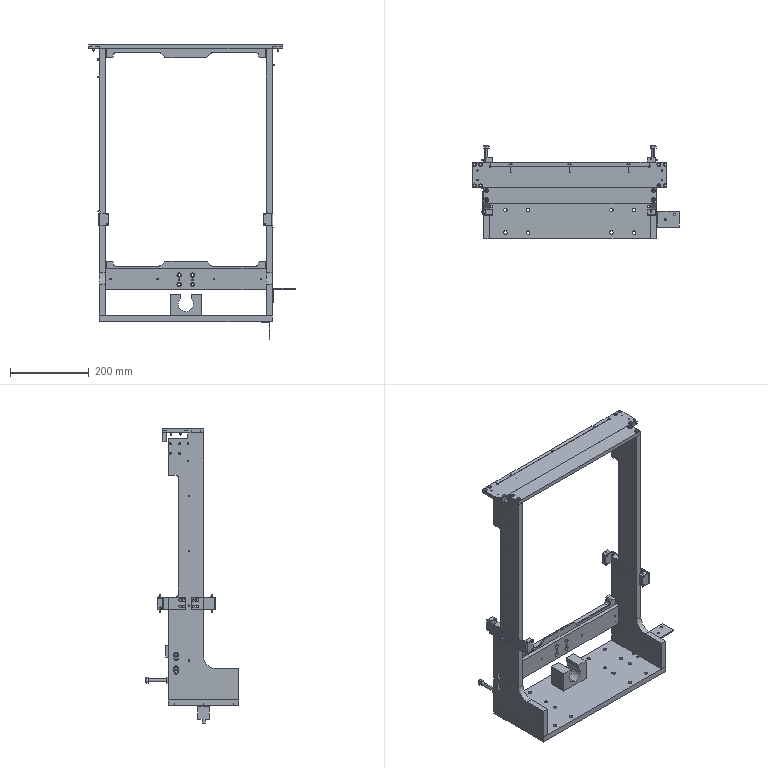Assembly | SolidWorks | mm | 33 component files | 33 solids | 1082 faces | box 526.5 x 239 x 749 mm | volume 4007622 mm3 | cylinder 498 | plane 446 | cone 118 | sphere 20 | commonest cylinder face diameters 5 x69 6.6 x50 11 x47 10 x42 9 x40 3.3 x32 3 x32 5.5 x24
Bill of materials:
30-20A | 1 |  | Flat rectangular plate with many through-holes in a symmetric pattern.
30-24A | 1 |  | Rectangular block with a U-shaped slot: a round bore runs through the block and opens to the top face through a straight-sided slot.
30-27A | 1 |  | Tall, thin, roughly L-shaped plate: a long vertical upright with a short foot at the bottom joined by a rounded inside corner, a long relief cut along one edge, and scattered holes.
30-28A | 1 |  | Tall, thin, roughly L-shaped plate almost identical to unnamed part, with a different hole pattern: smaller holes at the top and two extra small holes in the foot.
30-29A | 1 |  | Long, thin, flat bar with stepped ends: a raised tab at each end and hole groups at both ends, including slot-like or notched openings at the edges.
30-30A | 1 |  | Plain, long, thin rectangular flat bar with two through-holes at each end.
30-32A | 1 |  | Long, narrow, bar-shaped plate with a shaped lower edge: a down-stepped foot at each end, a wide central lobe with angled sides, and three evenly spaced round holes along the upper area.
30-41A | 1 |  | Bent L-shaped bracket with a radiused bend: a longer flange with two holes and a shorter flange at right angles with two holes.
30-49A | 4 |  | Thin L-shaped bracket with a radiused bend: one flange has two elongated slots, the other has two round holes.
30-51A | 1 |  | Small bent bracket with a radiused bend: a horizontal flange with two round holes and a vertical flange ending in a narrower tab at the bottom.
KFQAPP3-P3.00-L4-B4.0 | 8 |  | Solid cylindrical pin with one hemispherical (domed) end and one flat end.
KFQAPP4-P4.00-L4-B4.0 | 2 |  | Solid cylindrical pin with one hemispherical (domed) end and one flat end.
30-31A | 1 |  | Long, thin rectangular flat bar with a pattern of small and larger through holes across its broad face, plus two holes in one end face.
30-33A | 1 |  | Long rectangular bar with a stepped top profile: a raised tab at each end with a small hooked notch, lower recessed runs, and a raised center section with angled transitions; two through holes in the center region.
Q20EBanner | 2 |  | Rectangular block body with two through holes near opposite corners, an angled cylindrical protrusion leaving one corner, a small cylindrical stub on one face, and two shallow raised rectangular pads on one side face.
Q20NRBanner | 2 |  | Rectangular block body with two through holes, an angled cylindrical protrusion from a chamfered corner, and small raised pads on one side face; close to a mirrored or reoriented version of the previous block part.
NUT_K8 | 2 |  | Hexagonal nut-like body with a central round bore and chamfered corners on both faces.
UST8_60b | 2 |  | Hex-head bolt-like part: a hexagonal head with a short cylindrical boss on its outer face and a long plain cylindrical shank ending in a chamfered tip.
Mates:
1. coincident | 30-20A-1 face at (-869.208, 12.908, 39.188) dir (0, 0, 1) | 30-28A-1 face at (-444.208, -167.092, 39.188) dir (0, 0, -1)
2. coincident | 30-20A-1 face at (-429.208, -167.092, 24.188) dir (1, 0, 0) | 30-28A-1 face at (-429.208, -107.092, 149.188) dir (1, 0, 0)
3. coincident | 30-20A-1 face at (-869.208, -167.092, 24.188) dir (0, -1, 0) | 30-28A-1 face at (-444.208, -167.092, 39.188) dir (0, -1, 0)
4. coincident | 30-20A-1 face at (-869.208, 12.908, 39.188) dir (0, 0, 1) | 30-27A-1 face at (-869.208, -167.092, 39.188) dir (0, 0, -1)
5. coincident | 30-20A-1 face at (-869.208, -167.092, 24.188) dir (-1, 0, 0) | 30-27A-1 face at (-869.208, -107.092, 149.188) dir (-1, 0, 0)
6. coincident | 30-20A-1 face at (-869.208, 12.908, 24.188) dir (0, 1, 0) | 30-27A-1 face at (-869.208, 12.908, 39.188) dir (0, 1, 0)
7. coincident | 30-20A-1 plane at (-649.208, -77.092, 39.188) dir (1, 0, 0) | 30-24A-1 plane at (-649.208, -37.092, 66.188) dir (-1, 0, 0)
8. coincident | 30-20A-1 plane at (-649.208, -77.092, 39.188) dir (1, 0, 0) | assembly plane at (-649.208, 11.408, 176.688) dir (1, 0, 0)
9. distance | 30-28A-1 face at (-444.208, 12.908, 39.188) dir (0, 1, 0) | assembly face at (-224.366, 15.085, 546.382) dir (0, 1, 0)
10. distance | 30-28A-1 face at (-444.208, 12.908, 39.188) dir (0, 1, 0) | UST8_60-1/UST8_60b-1 face at (-859.001, 4.408, 90.956) dir (0, -1, 0)
11. concentric | 30-27A-1 face at (-861.708, 12.908, 89.188) dir (0, 1, 0) r 4.05 | UST8_60-1/UST8_60b-1 face at (-861.708, 4.408, 89.188) dir (0, 1, 0) r 4
12. concentric | 30-28A-1 face at (-436.708, 12.908, 89.188) dir (0, 1, 0) r 4.05 | UST8_60-2/UST8_60b-1 face at (-436.708, 4.408, 89.188) dir (0, 1, 0) r 4
13. distance | 30-28A-1 face at (-444.208, 12.908, 39.188) dir (0, 1, 0) | UST8_60-2/NUT_K8-1 face at (-436.708, 12.908, 89.188) dir (0, -1, 0)
14. coincident | 30-28A-1 face at (-429.208, -107.092, 149.188) dir (1, 0, 0) | assembly face at (-419.208, -53.092, 330.922) dir (-1, 0, 0)
15. coincident | 30-28A-1 face at (-444.208, -77.092, 719.188) dir (0, -1, 0) | assembly face at (-417.208, -51.092, 330.922) dir (0, 1, 0)
16. concentric | 30-27A-1 face at (-861.708, -45.092, 719.188) dir (0, 0, 1) r 2.5 | 30-30A-1 face at (-861.708, -45.092, 729.188) dir (0, 0, 1) r 5.5
17. concentric | 30-27A-1 face at (-861.708, -69.092, 719.188) dir (0, 0, 1) r 2.5 | 30-30A-1 face at (-861.708, -69.092, 729.188) dir (0, 0, 1) r 5.5
18. coincident | 30-27A-1 face at (-869.208, 12.908, 719.188) dir (0, 0, 1) | 30-30A-1 face at (-869.208, -77.092, 719.188) dir (0, 0, -1)
19. concentric | 30-27A-1 face at (-854.208, -37.592, 692.188) dir (-1, 0, 0) r 1.5 | KFQAPP3-P3.00-L4-B4.0-1 face at (-908.289, -37.592, 692.188) dir (-1, 0, 0) r 1.5
20. concentric | 30-27A-1 face at (-854.208, -37.592, 647.188) dir (-1, 0, 0) r 1.5 | KFQAPP3-P3.00-L4-B4.0-2 face at (-908.289, -37.592, 647.188) dir (-1, 0, 0) r 1.5
21. coincident | KFQAPP3-P3.00-L4-B4.0-2 face at (-865.208, -37.996, 648.632) dir (1, 0, 0) | KFQAPP3-P3.00-L4-B4.0-1 face at (-865.208, -37.952, 693.644) dir (1, 0, 0)
22. concentric | 30-28A-1 face at (-444.208, 7.908, 679.188) dir (1, 0, 0) r 1.5 | KFQAPP3-P3.00-L4-B4.0-7 face at (-390.126, 7.908, 679.188) dir (1, 0, 0) r 1.5
23. concentric | 30-28A-1 face at (-444.208, -16.092, 679.188) dir (1, 0, 0) r 1.5 | KFQAPP3-P3.00-L4-B4.0-8 face at (-390.126, -16.092, 679.188) dir (1, 0, 0) r 1.5
24. concentric | MGPM25-20Z-A93LAssembly-1/30-31A-1 face at (-632.208, -22.092, 131.188) dir (0, 1, 0) r 2 | KFQAPP4-P4.00-L4-B4.0-1 face at (-632.208, 37.24, 131.188) dir (0, 1, 0) r 2
25. concentric | MGPM25-20Z-A93LAssembly-1/30-31A-1 face at (-666.208, -22.092, 131.188) dir (0, 1, 0) r 2 | KFQAPP4-P4.00-L4-B4.0-2 face at (-666.208, 37.24, 131.188) dir (0, 1, 0) r 2
26. coincident | KFQAPP4-P4.00-L4-B4.0-2 face at (-664.285, -6.092, 130.637) dir (0, -1, 0) | KFQAPP4-P4.00-L4-B4.0-1 face at (-631.277, -6.092, 129.418) dir (0, -1, 0)
27. concentric | 30-29A-1 face at (-884.208, 5.908, 719.188) dir (0, 0, 1) r 1.5 | KFQAPP3-P3.00-L4-B4.0-3 face at (-884.208, 5.908, 680.106) dir (0, 0, -1) r 1.5
28. concentric | 30-29A-1 face at (-884.208, -18.092, 719.188) dir (0, 0, 1) r 1.5 | KFQAPP3-P3.00-L4-B4.0-4 face at (-884.208, -18.092, 680.106) dir (0, 0, -1) r 1.5
29. coincident | KFQAPP3-P3.00-L4-B4.0-3 face at (-884.901, 7.239, 723.188) dir (0, 0, 1) | KFQAPP3-P3.00-L4-B4.0-4 face at (-883.734, -16.668, 723.188) dir (0, 0, 1)
30. concentric | 30-29A-1 face at (-414.208, 5.908, 719.188) dir (0, 0, 1) r 1.5 | KFQAPP3-P3.00-L4-B4.0-5 face at (-414.208, 5.908, 680.106) dir (0, 0, -1) r 1.5
31. concentric | 30-29A-1 face at (-414.208, -18.092, 719.188) dir (0, 0, 1) r 1.5 | KFQAPP3-P3.00-L4-B4.0-6 face at (-414.208, -18.092, 680.106) dir (0, 0, -1) r 1.5
32. coincident | KFQAPP3-P3.00-L4-B4.0-5 face at (-415.412, 6.803, 723.188) dir (0, 0, 1) | KFQAPP3-P3.00-L4-B4.0-3 face at (-884.901, 7.239, 723.188) dir (0, 0, 1)
33. coincident | KFQAPP3-P3.00-L4-B4.0-6 face at (-415.384, -17.161, 723.188) dir (0, 0, 1) | KFQAPP3-P3.00-L4-B4.0-5 face at (-415.412, 6.803, 723.188) dir (0, 0, 1)
34. coincident | 30-27A-1 face at (-869.208, -107.092, 149.188) dir (-1, 0, 0) | 30-49A-1 face at (-869.208, 27.908, 269.188) dir (1, 0, 0)
35. coincident | 30-27A-1 face at (-869.208, -107.092, 149.188) dir (-1, 0, 0) | 30-49A-2 face at (-869.208, -107.092, 301.188) dir (1, 0, 0)
36. coincident | 30-49A-1 face at (-868.208, 25.908, 269.188) dir (0, 0, -1) | 30-49A-2 face at (-868.208, -104.092, 269.188) dir (0, 0, -1)
37. distance | 30-27A-1 face at (-869.208, -77.092, 719.188) dir (0, -1, 0) | 30-49A-2 face at (-871.208, -47.092, 301.188) dir (0, 1, 0)
38. coincident | 30-28A-1 face at (-429.208, -107.092, 149.188) dir (1, 0, 0) | 30-49A-3 face at (-429.208, 27.908, 301.188) dir (-1, 0, 0)
39. coincident | 30-28A-1 face at (-429.208, -107.092, 149.188) dir (1, 0, 0) | 30-49A-4 face at (-429.208, -107.092, 269.188) dir (-1, 0, 0)
40. distance | 30-28A-1 face at (-444.208, -77.092, 719.188) dir (0, -1, 0) | 30-49A-4 face at (-427.208, -47.092, 269.188) dir (0, 1, 0)
41. coincident | 30-49A-3 face at (-430.208, 25.908, 301.188) dir (0, 0, 1) | 30-49A-4 face at (-430.208, -104.092, 301.188) dir (0, 0, 1)
42. concentric | 30-49A-1 face at (-850.208, 27.908, 272.488) dir (0, 1, 0) r 1.75 | Q20EBanner-1 face at (-850.208, 27.908, 272.488) dir (0, -1, 0) r 1.25
43. concentric | 30-49A-1 face at (-850.208, 27.908, 297.888) dir (0, 1, 0) r 1.75 | Q20EBanner-1 face at (-850.208, 27.908, 297.888) dir (0, -1, 0) r 1.25
44. coincident | 30-49A-1 face at (-846.208, 27.908, 269.188) dir (0, 1, 0) | Q20EBanner-1 face at (-846.908, 27.908, 269.188) dir (0, -1, 0)
45. concentric | 30-49A-3 face at (-448.208, 27.908, 297.888) dir (0, 1, 0) r 1.75 | Q20NRBanner-1 face at (-448.208, 27.908, 297.888) dir (0, -1, 0) r 1.25
46. concentric | 30-49A-3 face at (-448.208, 27.908, 272.488) dir (0, 1, 0) r 1.75 | Q20NRBanner-1 face at (-448.208, 27.908, 272.488) dir (0, -1, 0) r 1.25
47. coincident | 30-49A-3 face at (-452.208, 27.908, 301.188) dir (0, 1, 0) | Q20NRBanner-1 face at (-451.508, 27.908, 301.188) dir (0, -1, 0)
48. concentric | 30-49A-2 face at (-850.208, -107.092, 272.488) dir (0, -1, 0) r 1.75 | Q20EBanner-2 face at (-850.208, -105.092, 272.488) dir (0, -1, 0) r 1.25
49. concentric | 30-49A-2 face at (-850.208, -107.092, 297.888) dir (0, -1, 0) r 1.75 | Q20EBanner-2 face at (-850.208, -105.092, 297.888) dir (0, -1, 0) r 1.25
50. concentric | 30-49A-4 face at (-448.208, -107.092, 272.488) dir (0, -1, 0) r 1.75 | Q20NRBanner-2 face at (-448.208, -105.092, 272.488) dir (0, -1, 0) r 1.25
51. concentric | 30-49A-4 face at (-448.208, -107.092, 297.888) dir (0, -1, 0) r 1.75 | Q20NRBanner-2 face at (-448.208, -105.092, 297.888) dir (0, -1, 0) r 1.25
52. coincident | 30-28A-1 face at (-429.208, -107.092, 149.188) dir (1, 0, 0) | 30-41A-1 face at (-429.208, -97.092, 105.188) dir (-1, 0, 0)
53. distance | 30-28A-1 face at (-444.208, -107.092, 119.188) dir (0, 0, 1) | 30-41A-1 face at (-425.208, -97.092, 109.188) dir (0, 0, 1)
54. coincident | 30-49A-1 face at (-868.208, 24.908, 301.188) dir (0, 0, 1) | 30-49A-3 face at (-430.208, 25.908, 301.188) dir (0, 0, 1)
55. coincident | MGPM25-20Z-A93LAssembly-1/30-31A-1 face at (-856.208, -2.092, 160.188) dir (-1, 0, 0) | 30-27A-1 face at (-856.208, -10.092, 165.688) dir (1, 0, 0)
56. coincident | 30-20A-1 face at (-869.208, 12.908, 39.188) dir (0, 0, 1) | 30-24A-1 face at (-609.208, -59.592, 39.188) dir (0, 0, -1)
57. distance | MGPM25-20Z-A93LAssembly-1/30-31A-1 face at (-442.208, -2.092, 160.188) dir (0, 1, 0) | 30-28A-1 face at (-444.208, 12.908, 39.188) dir (0, 1, 0)
58. distance | 30-27A-1 face at (-869.208, 12.908, 39.188) dir (0, 1, 0) | 30-49A-1 face at (-871.208, -32.092, 269.188) dir (0, -1, 0)
59. coincident | Q20EBanner-1 face at (-846.908, 39.908, 269.188) dir (0, 1, 0) | Q20NRBanner-1 face at (-451.508, 39.908, 301.188) dir (0, 1, 0)
60. coincident | 30-20A-1 face at (-869.208, 12.908, 24.188) dir (0, 0, -1) | 30-51A-1 face at (-437.208, -92.092, 24.188) dir (0, 0, 1)
61. coincident | 30-49A-4 face at (-452.208, -105.092, 269.188) dir (0, 1, 0) | Q20NRBanner-2 face at (-451.508, -105.092, 301.188) dir (0, -1, 0)
62. coincident | 30-49A-2 face at (-846.208, -105.092, 301.188) dir (0, 1, 0) | Q20EBanner-2 face at (-846.908, -105.092, 269.188) dir (0, -1, 0)
63. distance | 30-28A-1 face at (-444.208, -167.092, 39.188) dir (0, -1, 0) | 30-41A-1 face at (-424.208, -137.092, 104.188) dir (0, -1, 0)
64. coincident | 30-29A-1 face at (-896.708, -37.092, 729.188) dir (0, 0, 1) | 30-32A-1 face at (-851.708, 16.908, 729.188) dir (0, 0, 1)
65. width | 30-32A-1 face at (-851.708, 26.908, 729.188) dir (-1, 0, 0) | 30-32A-1 face at (-446.708, 26.908, 729.188) dir (1, 0, 0) | 30-29A-1 face at (-896.708, 26.908, 729.188) dir (-1, 0, 0) | 30-29A-1 face at (-401.708, 26.908, 729.188) dir (1, 0, 0)
66. coincident | 30-29A-1 face at (-851.708, 16.908, 719.188) dir (0, 1, 0) | 30-32A-1 face at (-851.708, 16.908, 729.188) dir (0, -1, 0)
67. distance | 30-20A-1 face at (-869.208, 12.908, 24.188) dir (0, 0, -1) | assembly face at (-649.208, 18.908, 102.688) dir (0, 0, -1)
68. concentric | 30-20A-1 face at (-616.708, -22.092, 24.188) dir (0, 0, -1) r 4.5 | 30-24A-1 face at (-616.708, -22.092, 39.188) dir (0, 0, -1) r 3.4
69. coincident | 30-27A-1 face at (-854.208, 12.908, 301.188) dir (0, 0, 1) | 30-49A-1 face at (-868.208, 24.908, 301.188) dir (0, 0, 1)
70. concentric | 30-20A-1 face at (-449.208, -69.592, 24.188) dir (0, 0, -1) r 2.5 | 30-51A-1 face at (-449.208, -69.592, 24.188) dir (0, 0, -1) r 3.5
71. concentric | 30-20A-1 face at (-449.208, -84.592, 24.188) dir (0, 0, -1) r 2.5 | 30-51A-1 face at (-449.208, -84.592, 24.188) dir (0, 0, -1) r 3.5
72. distance | 30-27A-1 face at (-869.208, -107.092, 149.188) dir (-1, 0, 0) | KFQAPP3-P3.00-L4-B4.0-1 face at (-865.208, -37.952, 693.644) dir (1, 0, 0)
73. distance | 30-29A-1 face at (-896.708, -37.092, 719.188) dir (0, 0, -1) | KFQAPP3-P3.00-L4-B4.0-3 face at (-884.901, 7.239, 723.188) dir (0, 0, 1)
74. distance | 30-28A-1 face at (-429.208, -107.092, 149.188) dir (1, 0, 0) | KFQAPP3-P3.00-L4-B4.0-7 face at (-433.208, 8.89, 680.322) dir (-1, 0, 0)
75. coincident | KFQAPP3-P3.00-L4-B4.0-7 face at (-433.208, 8.89, 680.322) dir (-1, 0, 0) | KFQAPP3-P3.00-L4-B4.0-8 face at (-433.208, -14.596, 679.072) dir (-1, 0, 0)
76. distance | MGPM25-20Z-A93LAssembly-1/30-31A-1 face at (-442.208, -2.092, 160.188) dir (0, 1, 0) | KFQAPP4-P4.00-L4-B4.0-1 face at (-631.277, -6.092, 129.418) dir (0, -1, 0)
77. coincident | 30-29A-1 face at (-896.708, -37.092, 729.188) dir (0, -1, 0) | 30-30A-1 face at (-869.208, -37.092, 729.188) dir (0, 1, 0)
78. coincident | 30-29A-1 face at (-896.708, -37.092, 729.188) dir (0, 0, 1) | 30-30A-1 face at (-869.208, -77.092, 729.188) dir (0, 0, 1)
79. coincident | 30-33A-1 face at (-103.417, 85.917, 179.823) dir (0, -1, 0) | 30-31A-1 face at (282.869, 85.917, 191.823) dir (0, 1, 0)
80. coincident | 30-33A-1 face at (-86.417, 89.917, 191.823) dir (0, 0, 1) | 30-31A-1 face at (282.869, 85.917, 191.823) dir (0, 0, 1)
81. distance | UST8_60b-1 plane at (30, 0, 0) dir (1, 0, 0) | NUT_K8-1 plane at (49, 0, 0) dir (-1, 0, 0)
82. coincident | UST8_60b-1 axis at (80.9, 0, 0) dir (-1, 0, 0) | NUT_K8-1 axis at (-31.9, 0, 0) dir (1, 0, 0)
83. angle | UST8_60b-1 plane at (0, 0, 0) dir (0, 0, -1) | NUT_K8-1 plane at (49, 0, 0) dir (0, 0, -1)